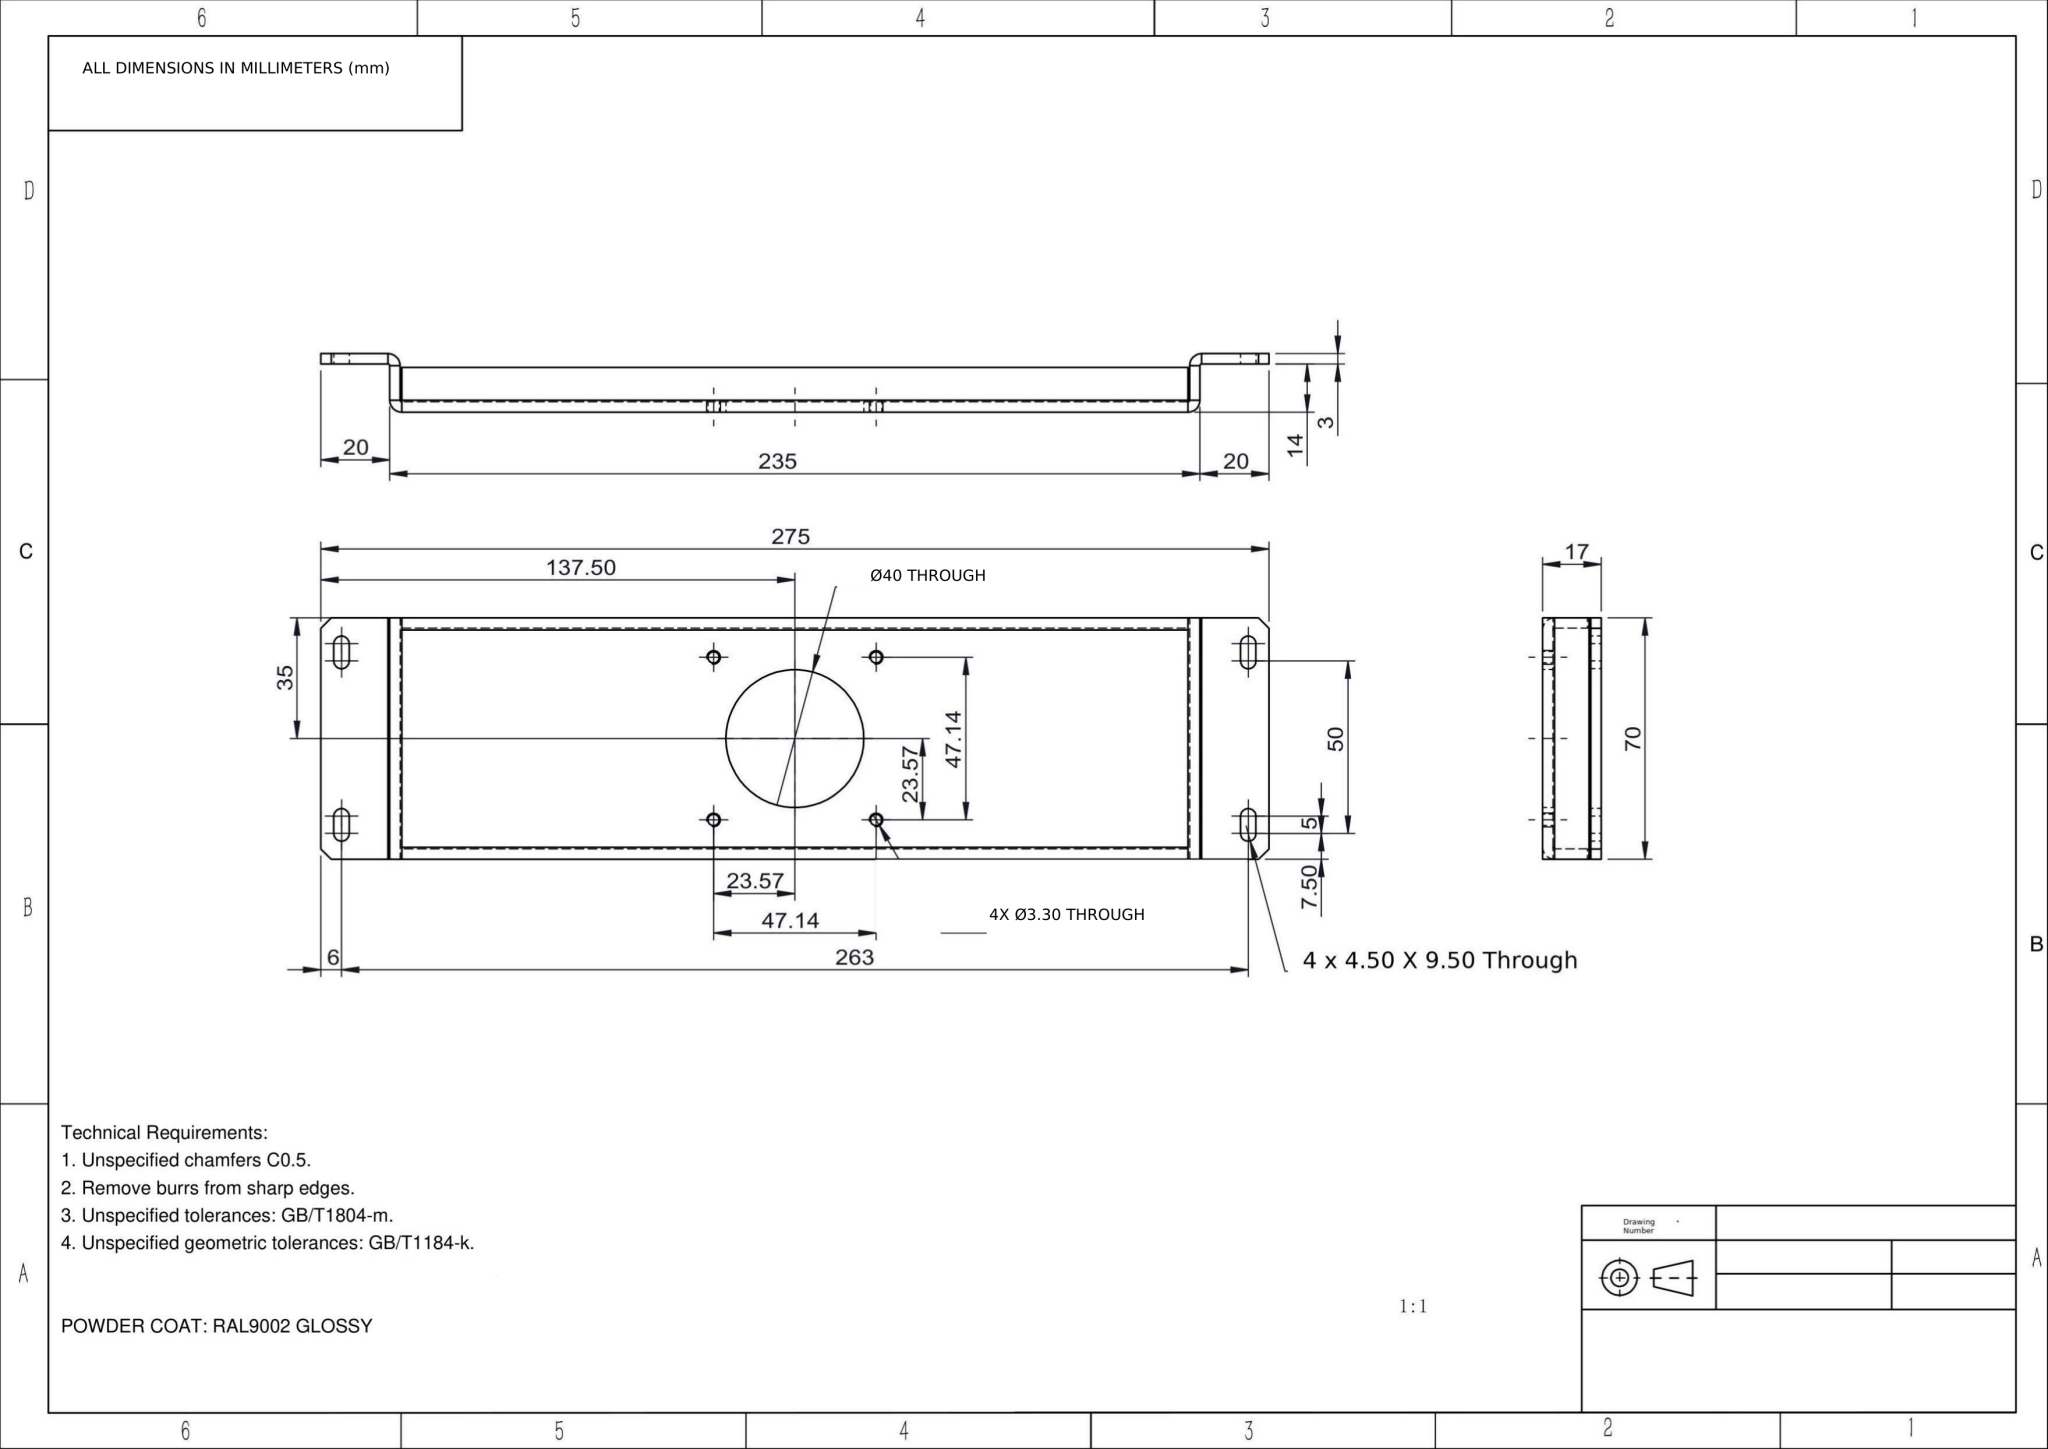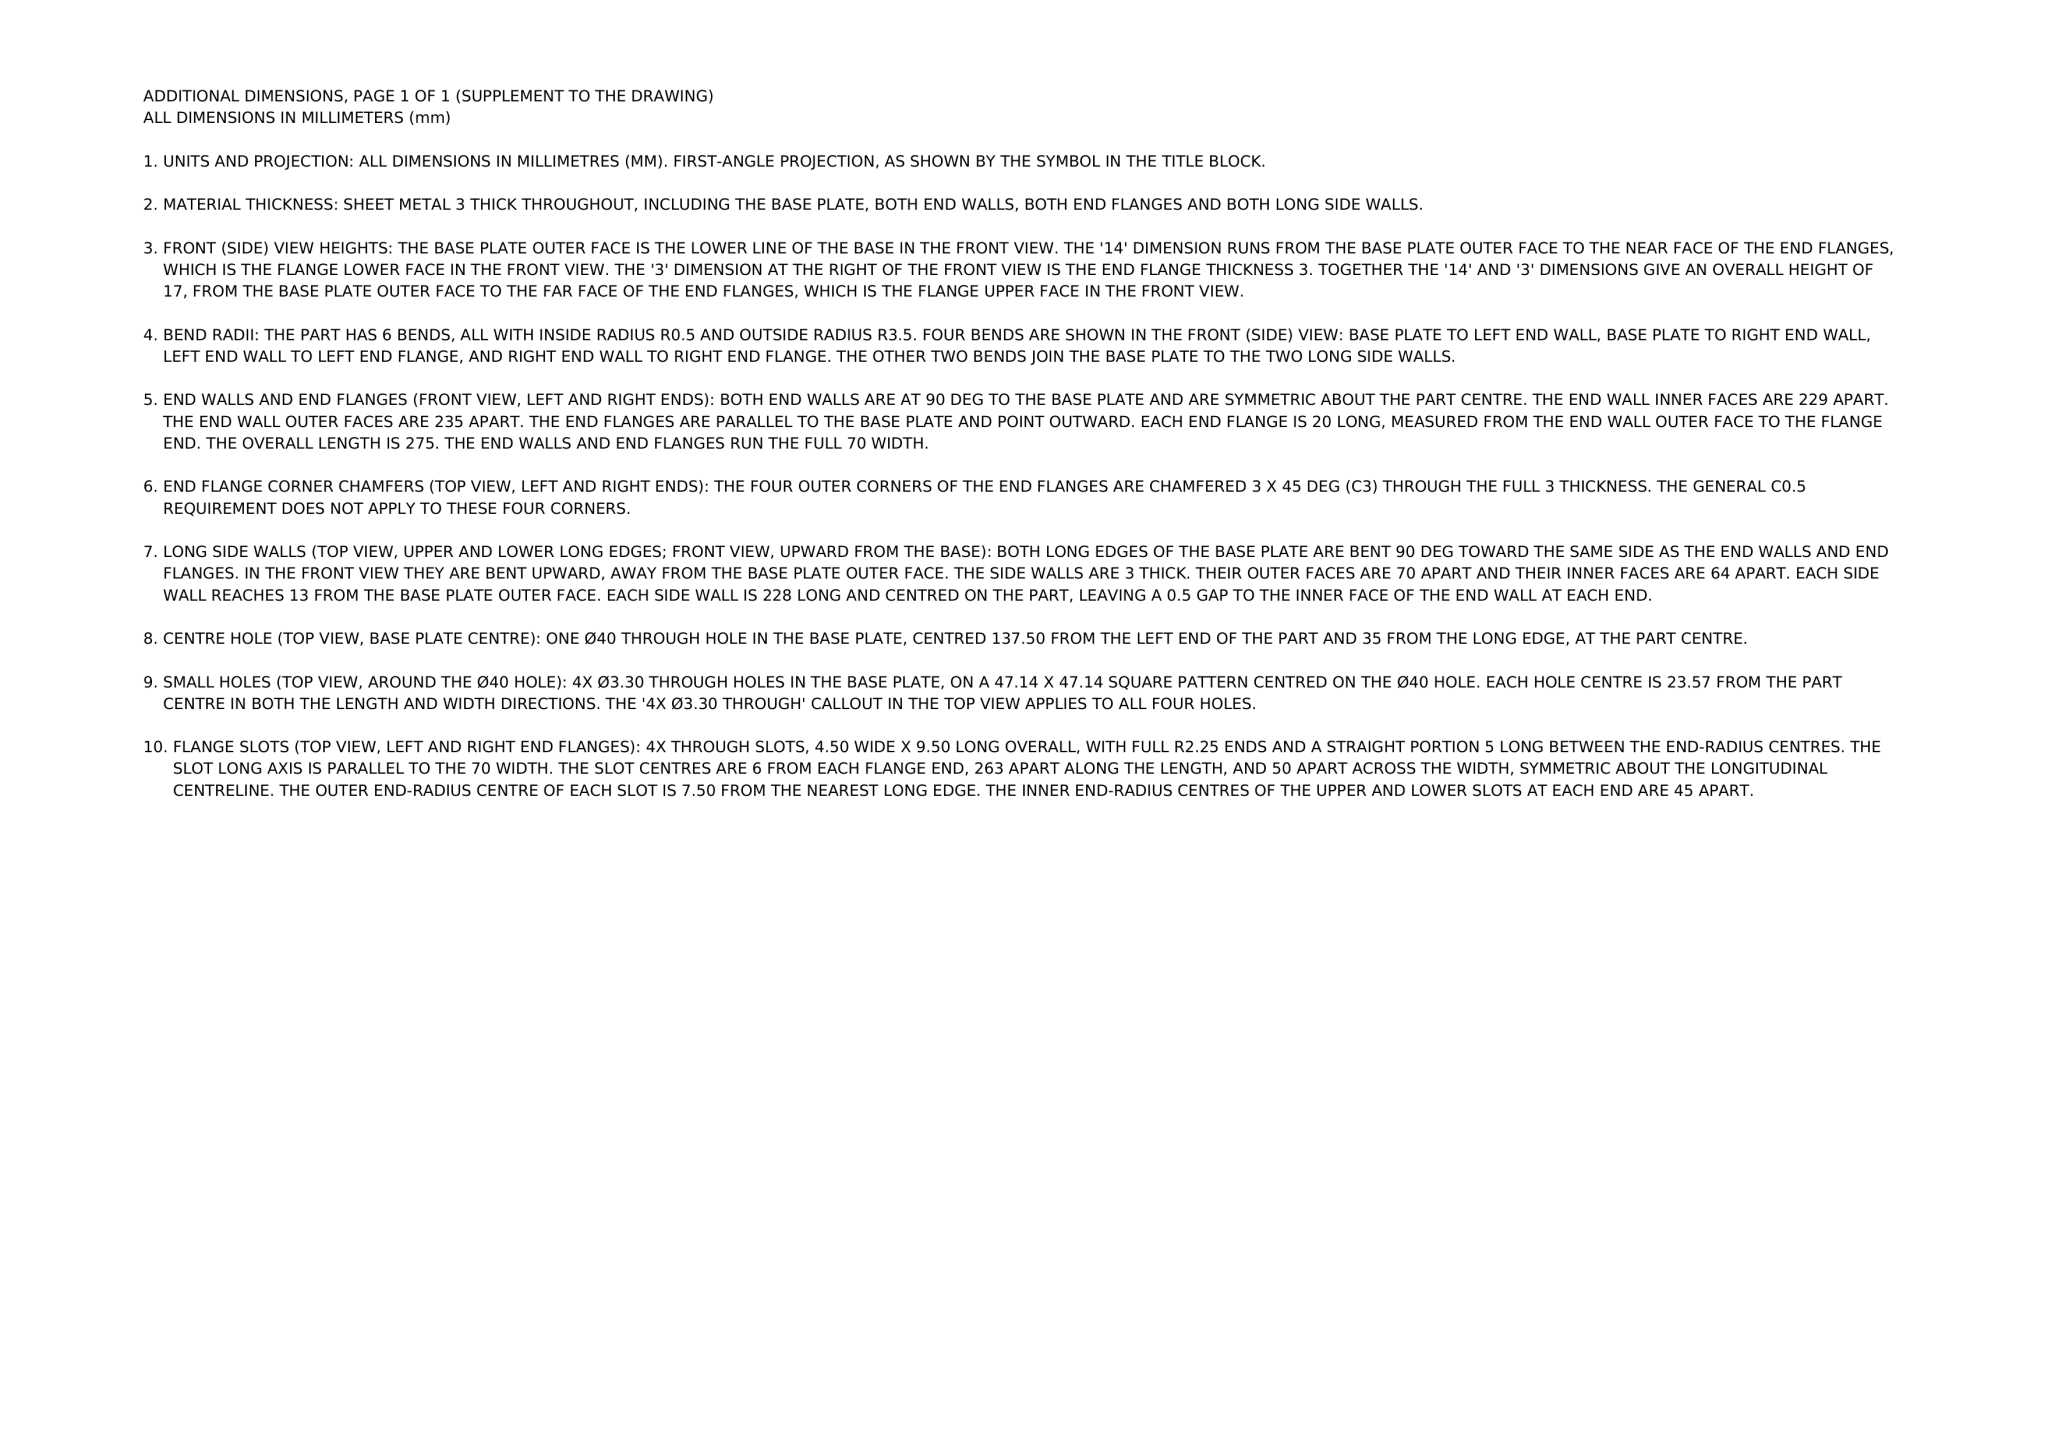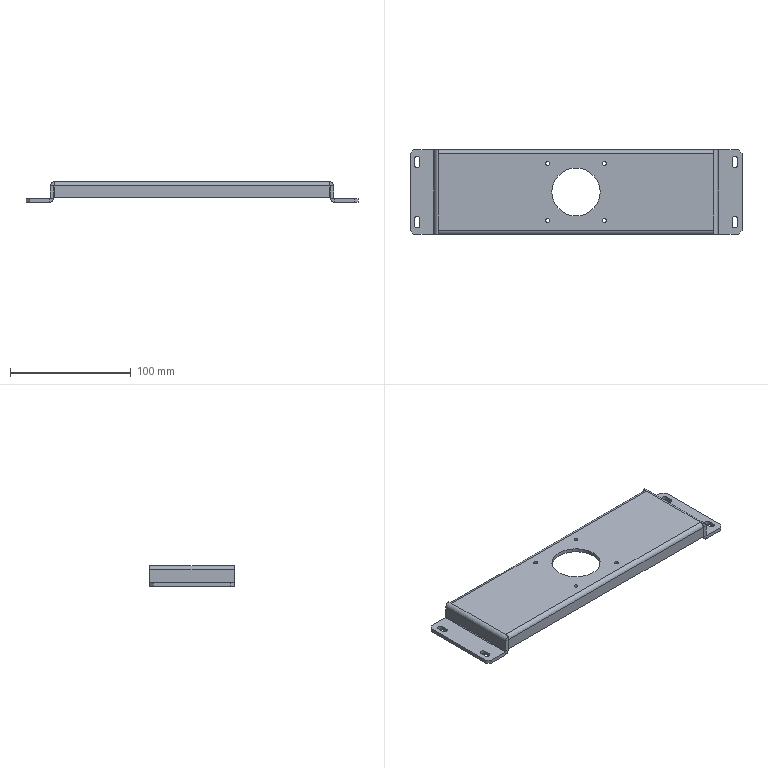Part | NX | mm | 1 solid | 88 faces | box 275 x 70 x 17 mm | volume 71027 mm3 | plane 58 | cylinder 30 | commonest cylinder face diameters 3.3 x8 4.5 x8 7 x6 1 x6 40 x2